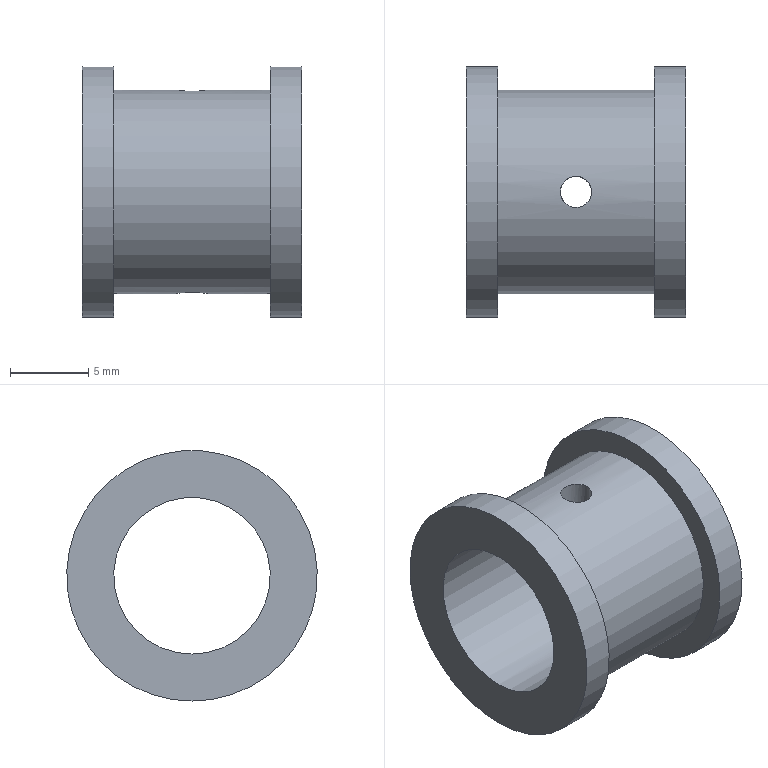Component | NX | 13__27_2 | 1 solid | 10 faces | volume 1023 mm3 | cylinder 6 | plane 4 | commonest cylinder face diameters 16 x2 2 x2 10 x1 13 x1